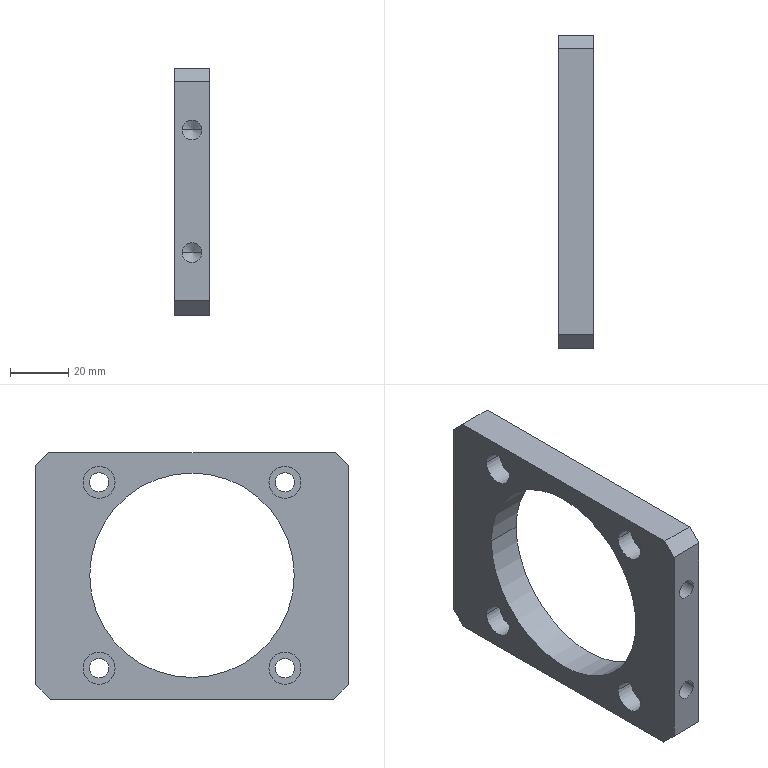Component | SolidWorks | 17081801-804-003A-1 | 1 solid | 48 faces | box 12 x 107 x 84.5 mm | volume 55606 mm3 | cylinder 26 | plane 14 | cone 8 | commonest cylinder face diameters 6.8 x8 11 x8 6.6 x8 70 x2 | material Q235
build123d program:
from build123d import *

# Parameters (mm, degrees)
SKETCH1_2_W                                     = 107
SKETCH1_2_H                                     = 85
SKETCH1_2_R                                     = 35
BOSS_EXTRUDE1_DEPTH                             = 6
M6_HEX_SOCKET_HEAD_CAP_SCREW_CBORE1_D           = 6.6
M6_HEX_SOCKET_HEAD_CAP_SCREW_CBORE1_CBORE_D     = 11
M6_HEX_SOCKET_HEAD_CAP_SCREW_CBORE1_CBORE_DEPTH = 6.4
CIRPATTERN1_COUNT                               = 4
CHAMFER1_SIZE                                   = 5
M8_TAPPED_HOLE1_D                               = 6.8
M8_TAPPED_HOLE1_DEPTH                           = 19.75
M8_TAPPED_HOLE1_TIP                             = 2.043
M8_TAPPED_HOLE2_D                               = 6.8
M8_TAPPED_HOLE2_DEPTH                           = 19.75
M8_TAPPED_HOLE2_TIP                             = 2.043
CUT_EXTRUDE1_DEPTH                              = 69.589
CUT_EXTRUDE1_DEPTH_BACK                         = 69.589
SKETCH1_W                                       = 120
SKETCH1_H                                       = 8


with BuildPart() as part:
    # Sketch1_2 → Boss-Extrude1 (new, symmetric)
    with BuildSketch(Plane.XY):
        Rectangle(SKETCH1_2_W, SKETCH1_2_H)
        Circle(SKETCH1_2_R, mode=Mode.SUBTRACT)
    extrude(amount=BOSS_EXTRUDE1_DEPTH, both=True)

    # M6 Hex Socket Head Cap Screw CBORE1 (through all)
    with Locations(Plane.XY.offset(6)):
        with Locations((31.82, 31.82)):
            m6_hex_socket_head_cap_screw_cbore1 = CounterBoreHole(M6_HEX_SOCKET_HEAD_CAP_SCREW_CBORE1_D / 2, M6_HEX_SOCKET_HEAD_CAP_SCREW_CBORE1_CBORE_D / 2, M6_HEX_SOCKET_HEAD_CAP_SCREW_CBORE1_CBORE_DEPTH)

    # CirPattern1: M6 Hex Socket Head Cap Screw CBORE1 ×4 about axis
    cirpattern1_axis = Axis((0, 0, 0), (0, 0, 1))
    for i in range(1, CIRPATTERN1_COUNT):
        add(m6_hex_socket_head_cap_screw_cbore1.rotate(cirpattern1_axis, i * 360 / CIRPATTERN1_COUNT), mode=Mode.SUBTRACT)

    # Chamfer1
    chamfer1_edges = [part.edges().sort_by_distance(p)[0] for p in [
        (-53.5, 42.5, 0),
        (53.5, 42.5, 0),
        (53.5, -42.5, 0),
        (-53.5, -42.5, 0),
    ]]
    chamfer(chamfer1_edges, length=CHAMFER1_SIZE)

    # M8 Tapped Hole1
    with Locations(Plane.ZY.offset(53.5)):
        with Locations((0, 21), (0, -21)):
            Hole(M8_TAPPED_HOLE1_D / 2, depth=M8_TAPPED_HOLE1_DEPTH)
            with Locations((0, 0, -(M8_TAPPED_HOLE1_DEPTH + M8_TAPPED_HOLE1_TIP / 2))):  # 118° drill point
                Cone(0, M8_TAPPED_HOLE1_D / 2, M8_TAPPED_HOLE1_TIP, mode=Mode.SUBTRACT)

    # M8 Tapped Hole2
    with Locations(Plane(origin=(53.5, 0, 0), x_dir=(0, 0, -1), z_dir=(1, 0, 0))):
        with Locations((0, 21), (0, -21)):
            Hole(M8_TAPPED_HOLE2_D / 2, depth=M8_TAPPED_HOLE2_DEPTH)
            with Locations((0, 0, -(M8_TAPPED_HOLE2_DEPTH + M8_TAPPED_HOLE2_TIP / 2))):  # 118° drill point
                Cone(0, M8_TAPPED_HOLE2_D / 2, M8_TAPPED_HOLE2_TIP, mode=Mode.SUBTRACT)

    # Sketch1 → Cut-Extrude1 (cut, two sides: drawn at the far end of the back side and taken through both)
    with BuildSketch(Plane.XY.offset(-CUT_EXTRUDE1_DEPTH_BACK)):
        with Locations((0, 46)):
            Rectangle(SKETCH1_W, SKETCH1_H)
    extrude(amount=CUT_EXTRUDE1_DEPTH + CUT_EXTRUDE1_DEPTH_BACK, mode=Mode.SUBTRACT)


solid = part.part

# Placed as in the assembly
solid = solid.moved(Location((-61.9, 2034.4, 178), (90, -90, 0)))